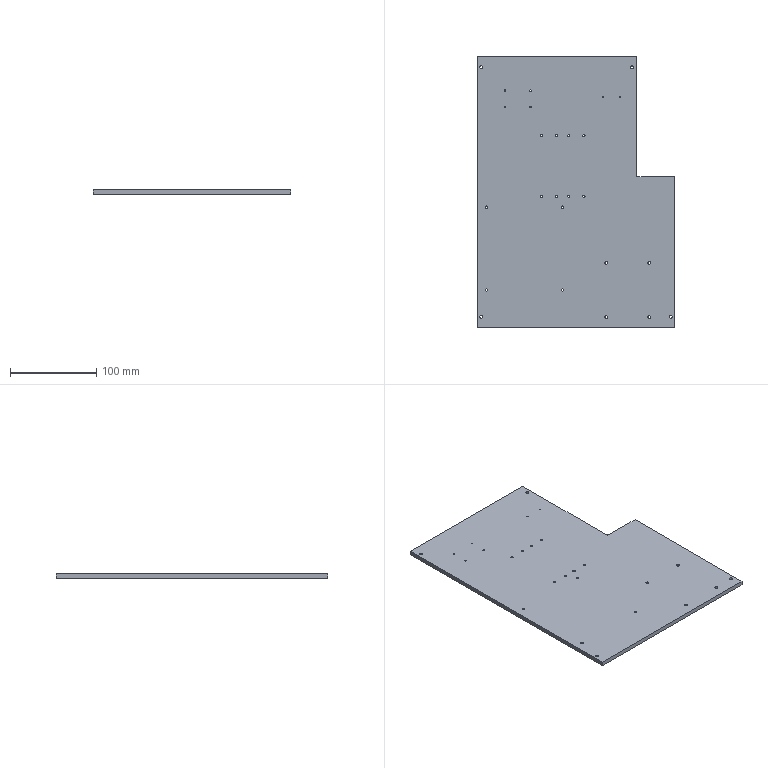CAM job | Mastercam | mm | 4 operations | part box 230 x 315.9 x 5
1. Contour (Ramp) | 4 - 4 平铣刀
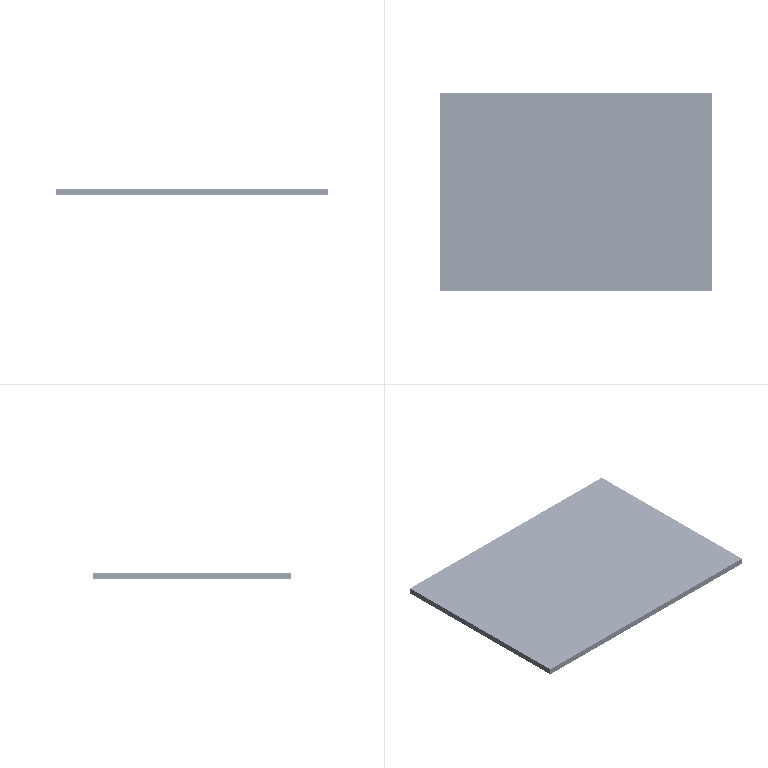2. Contour (2D) | 3 - 3 平铣刀
3. Drill/Counterbore | 5 - 4 倒角刀
4. Contour (2D chamfer) | 5 - 4 倒角刀